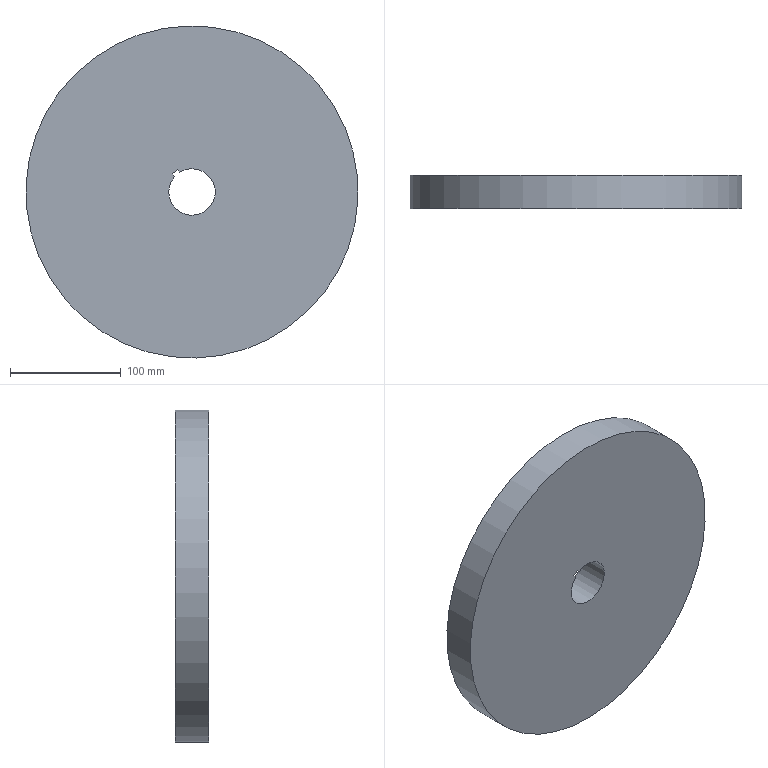Component | NX | MODEL1 | 1 solid | 7 faces | box 300 x 30 x 300 mm | volume 2078459 mm3 | plane 5 | cylinder 2 | commonest cylinder face diameters 300 x1 42 x1
STEP:
#1=CARTESIAN_POINT('',(0.,0.,0.));
#2=DIRECTION('',(0.,0.,1.));
#3=DIRECTION('',(1.,0.,0.));
#4=AXIS2_PLACEMENT_3D('',#1,#2,#3);
#5=CARTESIAN_POINT('',(844.342,50.431,-88.771));
#6=VERTEX_POINT('',#5);
#7=CARTESIAN_POINT('',(842.275,50.431,-86.308));
#8=VERTEX_POINT('',#7);
#9=CARTESIAN_POINT('',(844.342,50.431,-88.771));
#10=DIRECTION('',(-0.6428,0.,0.766));
#11=VECTOR('',#10,1.);
#12=LINE('',#9,#11);
#13=CARTESIAN_POINT('',(844.342,20.431,-88.771));
#14=DIRECTION('',(-0.766,0.,-0.6428));
#15=DIRECTION('',(0.6428,0.,-0.766));
#16=AXIS2_PLACEMENT_3D('',#13,#14,#15);
#17=PLANE('',#16);
#18=CARTESIAN_POINT('',(0.,-30.));
#19=DIRECTION('',(-1.,0.));
#20=VECTOR('',#19,1.);
#21=LINE('',#18,#20);
#22=(GEOMETRIC_REPRESENTATION_CONTEXT(2)PARAMETRIC_REPRESENTATION_CONTEXT()REPRESENTATION_CONTEXT('',''));
#23=DEFINITIONAL_REPRESENTATION('',(#21),#22);
#24=PCURVE('',#17,#23);
#25=CARTESIAN_POINT('',(860.,50.431,-102.764));
#26=DIRECTION('',(0.,-1.,0.));
#27=DIRECTION('',(0.766,0.,0.6428));
#28=AXIS2_PLACEMENT_3D('',#25,#26,#27);
#29=PLANE('',#28);
#30=CARTESIAN_POINT('',(-3.,20.785));
#31=DIRECTION('',(0.,1.));
#32=VECTOR('',#31,1.);
#33=LINE('',#30,#32);
#34=(GEOMETRIC_REPRESENTATION_CONTEXT(2)PARAMETRIC_REPRESENTATION_CONTEXT()REPRESENTATION_CONTEXT('',''));
#35=DEFINITIONAL_REPRESENTATION('',(#33),#34);
#36=PCURVE('',#29,#35);
#37=SURFACE_CURVE('',#12,(#24,#36),.PCURVE_S1.);
#38=EDGE_CURVE('',#6,#8,#37,.T.);
#39=ORIENTED_EDGE('',*,*,#38,.T.);
#40=CARTESIAN_POINT('',(842.275,20.431,-86.308));
#41=VERTEX_POINT('',#40);
#42=CARTESIAN_POINT('',(842.275,20.431,-86.308));
#43=DIRECTION('',(0.,1.,0.));
#44=VECTOR('',#43,1.);
#45=LINE('',#42,#44);
#46=CARTESIAN_POINT('',(-3.215,0.));
#47=DIRECTION('',(0.,-1.));
#48=VECTOR('',#47,1.);
#49=LINE('',#46,#48);
#50=(GEOMETRIC_REPRESENTATION_CONTEXT(2)PARAMETRIC_REPRESENTATION_CONTEXT()REPRESENTATION_CONTEXT('',''));
#51=DEFINITIONAL_REPRESENTATION('',(#49),#50);
#52=PCURVE('',#17,#51);
#53=CARTESIAN_POINT('',(842.275,20.431,-86.308));
#54=DIRECTION('',(-0.6428,0.,0.766));
#55=DIRECTION('',(-0.766,0.,-0.6428));
#56=AXIS2_PLACEMENT_3D('',#53,#54,#55);
#57=PLANE('',#56);
#58=CARTESIAN_POINT('',(0.,0.));
#59=DIRECTION('',(0.,-1.));
#60=VECTOR('',#59,1.);
#61=LINE('',#58,#60);
#62=(GEOMETRIC_REPRESENTATION_CONTEXT(2)PARAMETRIC_REPRESENTATION_CONTEXT()REPRESENTATION_CONTEXT('',''));
#63=DEFINITIONAL_REPRESENTATION('',(#61),#62);
#64=PCURVE('',#57,#63);
#65=SURFACE_CURVE('',#45,(#52,#64),.PCURVE_S1.);
#66=EDGE_CURVE('',#41,#8,#65,.T.);
#67=ORIENTED_EDGE('',*,*,#66,.F.);
#68=CARTESIAN_POINT('',(844.342,20.431,-88.771));
#69=VERTEX_POINT('',#68);
#70=CARTESIAN_POINT('',(844.342,20.431,-88.771));
#71=DIRECTION('',(-0.6428,0.,0.766));
#72=VECTOR('',#71,1.);
#73=LINE('',#70,#72);
#74=CARTESIAN_POINT('',(0.,0.));
#75=DIRECTION('',(-1.,0.));
#76=VECTOR('',#75,1.);
#77=LINE('',#74,#76);
#78=(GEOMETRIC_REPRESENTATION_CONTEXT(2)PARAMETRIC_REPRESENTATION_CONTEXT()REPRESENTATION_CONTEXT('',''));
#79=DEFINITIONAL_REPRESENTATION('',(#77),#78);
#80=PCURVE('',#17,#79);
#81=CARTESIAN_POINT('',(860.,20.431,-102.764));
#82=DIRECTION('',(0.,-1.,0.));
#83=DIRECTION('',(0.766,0.,0.6428));
#84=AXIS2_PLACEMENT_3D('',#81,#82,#83);
#85=PLANE('',#84);
#86=CARTESIAN_POINT('',(-3.,20.785));
#87=DIRECTION('',(0.,1.));
#88=VECTOR('',#87,1.);
#89=LINE('',#86,#88);
#90=(GEOMETRIC_REPRESENTATION_CONTEXT(2)PARAMETRIC_REPRESENTATION_CONTEXT()REPRESENTATION_CONTEXT('',''));
#91=DEFINITIONAL_REPRESENTATION('',(#89),#90);
#92=PCURVE('',#85,#91);
#93=SURFACE_CURVE('',#73,(#80,#92),.PCURVE_S1.);
#94=EDGE_CURVE('',#69,#41,#93,.T.);
#95=ORIENTED_EDGE('',*,*,#94,.F.);
#96=CARTESIAN_POINT('',(844.342,20.431,-88.771));
#97=DIRECTION('',(0.,1.,0.));
#98=VECTOR('',#97,1.);
#99=LINE('',#96,#98);
#100=CARTESIAN_POINT('',(0.,0.));
#101=DIRECTION('',(0.,-1.));
#102=VECTOR('',#101,1.);
#103=LINE('',#100,#102);
#104=(GEOMETRIC_REPRESENTATION_CONTEXT(2)PARAMETRIC_REPRESENTATION_CONTEXT()REPRESENTATION_CONTEXT('',''));
#105=DEFINITIONAL_REPRESENTATION('',(#103),#104);
#106=PCURVE('',#17,#105);
#107=CARTESIAN_POINT('',(860.,20.431,-102.764));
#108=DIRECTION('',(0.,1.,0.));
#109=DIRECTION('',(-0.766,0.,-0.6428));
#110=AXIS2_PLACEMENT_3D('',#107,#108,#109);
#111=CYLINDRICAL_SURFACE('',#110,21.);
#112=CARTESIAN_POINT('',(7.711,0.));
#113=DIRECTION('',(0.,1.));
#114=VECTOR('',#113,1.);
#115=LINE('',#112,#114);
#116=(GEOMETRIC_REPRESENTATION_CONTEXT(2)PARAMETRIC_REPRESENTATION_CONTEXT()REPRESENTATION_CONTEXT('',''));
#117=DEFINITIONAL_REPRESENTATION('',(#115),#116);
#118=PCURVE('',#111,#117);
#119=SURFACE_CURVE('',#99,(#106,#118),.PCURVE_S1.);
#120=EDGE_CURVE('',#69,#6,#119,.T.);
#121=ORIENTED_EDGE('',*,*,#120,.T.);
#122=EDGE_LOOP('',(#39,#67,#95,#121));
#123=FACE_BOUND('',#122,.T.);
#124=ADVANCED_FACE('',(#123),#17,.F.);
#125=CARTESIAN_POINT('',(846.871,50.431,-82.451));
#126=VERTEX_POINT('',#125);
#127=CARTESIAN_POINT('',(842.275,50.431,-86.308));
#128=DIRECTION('',(0.766,0.,0.6428));
#129=VECTOR('',#128,1.);
#130=LINE('',#127,#129);
#131=CARTESIAN_POINT('',(0.,-30.));
#132=DIRECTION('',(-1.,0.));
#133=VECTOR('',#132,1.);
#134=LINE('',#131,#133);
#135=(GEOMETRIC_REPRESENTATION_CONTEXT(2)PARAMETRIC_REPRESENTATION_CONTEXT()REPRESENTATION_CONTEXT('',''));
#136=DEFINITIONAL_REPRESENTATION('',(#134),#135);
#137=PCURVE('',#57,#136);
#138=CARTESIAN_POINT('',(-3.,24.));
#139=DIRECTION('',(1.,-0.));
#140=VECTOR('',#139,1.);
#141=LINE('',#138,#140);
#142=(GEOMETRIC_REPRESENTATION_CONTEXT(2)PARAMETRIC_REPRESENTATION_CONTEXT()REPRESENTATION_CONTEXT('',''));
#143=DEFINITIONAL_REPRESENTATION('',(#141),#142);
#144=PCURVE('',#29,#143);
#145=SURFACE_CURVE('',#130,(#137,#144),.PCURVE_S1.);
#146=EDGE_CURVE('',#8,#126,#145,.T.);
#147=ORIENTED_EDGE('',*,*,#146,.T.);
#148=CARTESIAN_POINT('',(846.871,20.431,-82.451));
#149=VERTEX_POINT('',#148);
#150=CARTESIAN_POINT('',(846.871,20.431,-82.451));
#151=DIRECTION('',(0.,1.,0.));
#152=VECTOR('',#151,1.);
#153=LINE('',#150,#152);
#154=CARTESIAN_POINT('',(-6.,0.));
#155=DIRECTION('',(0.,-1.));
#156=VECTOR('',#155,1.);
#157=LINE('',#154,#156);
#158=(GEOMETRIC_REPRESENTATION_CONTEXT(2)PARAMETRIC_REPRESENTATION_CONTEXT()REPRESENTATION_CONTEXT('',''));
#159=DEFINITIONAL_REPRESENTATION('',(#157),#158);
#160=PCURVE('',#57,#159);
#161=CARTESIAN_POINT('',(846.871,20.431,-82.451));
#162=DIRECTION('',(0.766,0.,0.6428));
#163=DIRECTION('',(-0.6428,0.,0.766));
#164=AXIS2_PLACEMENT_3D('',#161,#162,#163);
#165=PLANE('',#164);
#166=CARTESIAN_POINT('',(-0.,0.));
#167=DIRECTION('',(0.,-1.));
#168=VECTOR('',#167,1.);
#169=LINE('',#166,#168);
#170=(GEOMETRIC_REPRESENTATION_CONTEXT(2)PARAMETRIC_REPRESENTATION_CONTEXT()REPRESENTATION_CONTEXT('',''));
#171=DEFINITIONAL_REPRESENTATION('',(#169),#170);
#172=PCURVE('',#165,#171);
#173=SURFACE_CURVE('',#153,(#160,#172),.PCURVE_S1.);
#174=EDGE_CURVE('',#149,#126,#173,.T.);
#175=ORIENTED_EDGE('',*,*,#174,.F.);
#176=CARTESIAN_POINT('',(842.275,20.431,-86.308));
#177=DIRECTION('',(0.766,0.,0.6428));
#178=VECTOR('',#177,1.);
#179=LINE('',#176,#178);
#180=CARTESIAN_POINT('',(0.,0.));
#181=DIRECTION('',(-1.,0.));
#182=VECTOR('',#181,1.);
#183=LINE('',#180,#182);
#184=(GEOMETRIC_REPRESENTATION_CONTEXT(2)PARAMETRIC_REPRESENTATION_CONTEXT()REPRESENTATION_CONTEXT('',''));
#185=DEFINITIONAL_REPRESENTATION('',(#183),#184);
#186=PCURVE('',#57,#185);
#187=CARTESIAN_POINT('',(-3.,24.));
#188=DIRECTION('',(1.,-0.));
#189=VECTOR('',#188,1.);
#190=LINE('',#187,#189);
#191=(GEOMETRIC_REPRESENTATION_CONTEXT(2)PARAMETRIC_REPRESENTATION_CONTEXT()REPRESENTATION_CONTEXT('',''));
#192=DEFINITIONAL_REPRESENTATION('',(#190),#191);
#193=PCURVE('',#85,#192);
#194=SURFACE_CURVE('',#179,(#186,#193),.PCURVE_S1.);
#195=EDGE_CURVE('',#41,#149,#194,.T.);
#196=ORIENTED_EDGE('',*,*,#195,.F.);
#197=ORIENTED_EDGE('',*,*,#66,.T.);
#198=EDGE_LOOP('',(#147,#175,#196,#197));
#199=FACE_BOUND('',#198,.T.);
#200=ADVANCED_FACE('',(#199),#57,.F.);
#201=CARTESIAN_POINT('',(848.938,50.431,-84.914));
#202=VERTEX_POINT('',#201);
#203=CARTESIAN_POINT('',(846.871,50.431,-82.451));
#204=DIRECTION('',(0.6428,0.,-0.766));
#205=VECTOR('',#204,1.);
#206=LINE('',#203,#205);
#207=CARTESIAN_POINT('',(0.,-30.));
#208=DIRECTION('',(-1.,0.));
#209=VECTOR('',#208,1.);
#210=LINE('',#207,#209);
#211=(GEOMETRIC_REPRESENTATION_CONTEXT(2)PARAMETRIC_REPRESENTATION_CONTEXT()REPRESENTATION_CONTEXT('',''));
#212=DEFINITIONAL_REPRESENTATION('',(#210),#211);
#213=PCURVE('',#165,#212);
#214=CARTESIAN_POINT('',(3.,24.));
#215=DIRECTION('',(0.,-1.));
#216=VECTOR('',#215,1.);
#217=LINE('',#214,#216);
#218=(GEOMETRIC_REPRESENTATION_CONTEXT(2)PARAMETRIC_REPRESENTATION_CONTEXT()REPRESENTATION_CONTEXT('',''));
#219=DEFINITIONAL_REPRESENTATION('',(#217),#218);
#220=PCURVE('',#29,#219);
#221=SURFACE_CURVE('',#206,(#213,#220),.PCURVE_S1.);
#222=EDGE_CURVE('',#126,#202,#221,.T.);
#223=ORIENTED_EDGE('',*,*,#222,.T.);
#224=CARTESIAN_POINT('',(848.938,20.431,-84.914));
#225=VERTEX_POINT('',#224);
#226=CARTESIAN_POINT('',(848.938,20.431,-84.914));
#227=DIRECTION('',(0.,1.,0.));
#228=VECTOR('',#227,1.);
#229=LINE('',#226,#228);
#230=CARTESIAN_POINT('',(-3.215,0.));
#231=DIRECTION('',(0.,-1.));
#232=VECTOR('',#231,1.);
#233=LINE('',#230,#232);
#234=(GEOMETRIC_REPRESENTATION_CONTEXT(2)PARAMETRIC_REPRESENTATION_CONTEXT()REPRESENTATION_CONTEXT('',''));
#235=DEFINITIONAL_REPRESENTATION('',(#233),#234);
#236=PCURVE('',#165,#235);
#237=CARTESIAN_POINT('',(1.714,0.));
#238=DIRECTION('',(0.,1.));
#239=VECTOR('',#238,1.);
#240=LINE('',#237,#239);
#241=(GEOMETRIC_REPRESENTATION_CONTEXT(2)PARAMETRIC_REPRESENTATION_CONTEXT()REPRESENTATION_CONTEXT('',''));
#242=DEFINITIONAL_REPRESENTATION('',(#240),#241);
#243=PCURVE('',#111,#242);
#244=SURFACE_CURVE('',#229,(#236,#243),.PCURVE_S1.);
#245=EDGE_CURVE('',#225,#202,#244,.T.);
#246=ORIENTED_EDGE('',*,*,#245,.F.);
#247=CARTESIAN_POINT('',(846.871,20.431,-82.451));
#248=DIRECTION('',(0.6428,0.,-0.766));
#249=VECTOR('',#248,1.);
#250=LINE('',#247,#249);
#251=CARTESIAN_POINT('',(0.,0.));
#252=DIRECTION('',(-1.,0.));
#253=VECTOR('',#252,1.);
#254=LINE('',#251,#253);
#255=(GEOMETRIC_REPRESENTATION_CONTEXT(2)PARAMETRIC_REPRESENTATION_CONTEXT()REPRESENTATION_CONTEXT('',''));
#256=DEFINITIONAL_REPRESENTATION('',(#254),#255);
#257=PCURVE('',#165,#256);
#258=CARTESIAN_POINT('',(3.,24.));
#259=DIRECTION('',(0.,-1.));
#260=VECTOR('',#259,1.);
#261=LINE('',#258,#260);
#262=(GEOMETRIC_REPRESENTATION_CONTEXT(2)PARAMETRIC_REPRESENTATION_CONTEXT()REPRESENTATION_CONTEXT('',''));
#263=DEFINITIONAL_REPRESENTATION('',(#261),#262);
#264=PCURVE('',#85,#263);
#265=SURFACE_CURVE('',#250,(#257,#264),.PCURVE_S1.);
#266=EDGE_CURVE('',#149,#225,#265,.T.);
#267=ORIENTED_EDGE('',*,*,#266,.F.);
#268=ORIENTED_EDGE('',*,*,#174,.T.);
#269=EDGE_LOOP('',(#223,#246,#267,#268));
#270=FACE_BOUND('',#269,.T.);
#271=ADVANCED_FACE('',(#270),#165,.F.);
#272=CARTESIAN_POINT('',(974.907,20.431,-6.346));
#273=VERTEX_POINT('',#272);
#274=CARTESIAN_POINT('',(860.,20.431,-102.764));
#275=DIRECTION('',(0.,-1.,0.));
#276=DIRECTION('',(0.766,0.,0.6428));
#277=AXIS2_PLACEMENT_3D('',#274,#275,#276);
#278=CIRCLE('',#277,150.);
#279=CARTESIAN_POINT('',(860.,20.431,-102.764));
#280=DIRECTION('',(0.,1.,0.));
#281=DIRECTION('',(-0.766,0.,-0.6428));
#282=AXIS2_PLACEMENT_3D('',#279,#280,#281);
#283=CYLINDRICAL_SURFACE('',#282,150.);
#284=CARTESIAN_POINT('',(9.425,0.));
#285=DIRECTION('',(-1.,0.));
#286=VECTOR('',#285,1.);
#287=LINE('',#284,#286);
#288=(GEOMETRIC_REPRESENTATION_CONTEXT(2)PARAMETRIC_REPRESENTATION_CONTEXT()REPRESENTATION_CONTEXT('',''));
#289=DEFINITIONAL_REPRESENTATION('',(#287),#288);
#290=PCURVE('',#283,#289);
#291=CARTESIAN_POINT('',(0.,0.));
#292=DIRECTION('',(1.,0.));
#293=AXIS2_PLACEMENT_2D('',#291,#292);
#294=CIRCLE('',#293,150.);
#295=(GEOMETRIC_REPRESENTATION_CONTEXT(2)PARAMETRIC_REPRESENTATION_CONTEXT()REPRESENTATION_CONTEXT('',''));
#296=DEFINITIONAL_REPRESENTATION('',(#294),#295);
#297=PCURVE('',#85,#296);
#298=SURFACE_CURVE('',#278,(#290,#297),.PCURVE_S1.);
#299=EDGE_CURVE('',#273,#273,#298,.T.);
#300=ORIENTED_EDGE('',*,*,#299,.F.);
#301=CARTESIAN_POINT('',(974.907,50.431,-6.346));
#302=VERTEX_POINT('',#301);
#303=CARTESIAN_POINT('',(974.907,20.431,-6.346));
#304=CARTESIAN_POINT('',(974.907,50.431,-6.346));
#305=B_SPLINE_CURVE_WITH_KNOTS('',1,(#303,#304),.UNSPECIFIED.,.F.,.F.,(2,2),(0.,30.),.PIECEWISE_BEZIER_KNOTS.);
#306=CARTESIAN_POINT('',(9.425,0.));
#307=DIRECTION('',(0.,1.));
#308=VECTOR('',#307,1.);
#309=LINE('',#306,#308);
#310=(GEOMETRIC_REPRESENTATION_CONTEXT(2)PARAMETRIC_REPRESENTATION_CONTEXT()REPRESENTATION_CONTEXT('',''));
#311=DEFINITIONAL_REPRESENTATION('',(#309),#310);
#312=PCURVE('',#283,#311);
#313=CARTESIAN_POINT('',(3.142,0.));
#314=DIRECTION('',(0.,1.));
#315=VECTOR('',#314,1.);
#316=LINE('',#313,#315);
#317=(GEOMETRIC_REPRESENTATION_CONTEXT(2)PARAMETRIC_REPRESENTATION_CONTEXT()REPRESENTATION_CONTEXT('',''));
#318=DEFINITIONAL_REPRESENTATION('',(#316),#317);
#319=PCURVE('',#283,#318);
#320=SEAM_CURVE('',#305,(#312,#319),.PCURVE_S1.);
#321=EDGE_CURVE('',#273,#302,#320,.T.);
#322=ORIENTED_EDGE('',*,*,#321,.T.);
#323=CARTESIAN_POINT('',(860.,50.431,-102.764));
#324=DIRECTION('',(0.,-1.,0.));
#325=DIRECTION('',(0.766,0.,0.6428));
#326=AXIS2_PLACEMENT_3D('',#323,#324,#325);
#327=CIRCLE('',#326,150.);
#328=CARTESIAN_POINT('',(9.425,30.));
#329=DIRECTION('',(-1.,0.));
#330=VECTOR('',#329,1.);
#331=LINE('',#328,#330);
#332=(GEOMETRIC_REPRESENTATION_CONTEXT(2)PARAMETRIC_REPRESENTATION_CONTEXT()REPRESENTATION_CONTEXT('',''));
#333=DEFINITIONAL_REPRESENTATION('',(#331),#332);
#334=PCURVE('',#283,#333);
#335=CARTESIAN_POINT('',(0.,0.));
#336=DIRECTION('',(1.,0.));
#337=AXIS2_PLACEMENT_2D('',#335,#336);
#338=CIRCLE('',#337,150.);
#339=(GEOMETRIC_REPRESENTATION_CONTEXT(2)PARAMETRIC_REPRESENTATION_CONTEXT()REPRESENTATION_CONTEXT('',''));
#340=DEFINITIONAL_REPRESENTATION('',(#338),#339);
#341=PCURVE('',#29,#340);
#342=SURFACE_CURVE('',#327,(#334,#341),.PCURVE_S1.);
#343=EDGE_CURVE('',#302,#302,#342,.T.);
#344=ORIENTED_EDGE('',*,*,#343,.T.);
#345=ORIENTED_EDGE('',*,*,#321,.F.);
#346=EDGE_LOOP('',(#300,#322,#344,#345));
#347=FACE_BOUND('',#346,.T.);
#348=ADVANCED_FACE('',(#347),#283,.T.);
#349=ORIENTED_EDGE('',*,*,#245,.F.);
#350=CARTESIAN_POINT('',(860.,20.431,-102.764));
#351=DIRECTION('',(0.,1.,0.));
#352=DIRECTION('',(0.766,0.,0.6428));
#353=AXIS2_PLACEMENT_3D('',#350,#351,#352);
#354=CIRCLE('',#353,21.);
#355=CARTESIAN_POINT('',(-3.142,0.));
#356=DIRECTION('',(1.,0.));
#357=VECTOR('',#356,1.);
#358=LINE('',#355,#357);
#359=(GEOMETRIC_REPRESENTATION_CONTEXT(2)PARAMETRIC_REPRESENTATION_CONTEXT()REPRESENTATION_CONTEXT('',''));
#360=DEFINITIONAL_REPRESENTATION('',(#358),#359);
#361=PCURVE('',#111,#360);
#362=CARTESIAN_POINT('',(21.,0.));
#363=CARTESIAN_POINT('',(21.,-36.373));
#364=CARTESIAN_POINT('',(-10.5,-18.187));
#365=CARTESIAN_POINT('',(-42.,-0.));
#366=CARTESIAN_POINT('',(-10.5,18.187));
#367=CARTESIAN_POINT('',(21.,36.373));
#368=CARTESIAN_POINT('',(21.,0.));
#369=(BOUNDED_CURVE()B_SPLINE_CURVE(2,(#362,#363,#364,#365,#366,#367,#368),.UNSPECIFIED.,.T.,.F.)B_SPLINE_CURVE_WITH_KNOTS((1,2,2,2,2,1),(-2.094,0.,2.094,4.189,6.283,8.378),.UNSPECIFIED.)CURVE()GEOMETRIC_REPRESENTATION_ITEM()RATIONAL_B_SPLINE_CURVE((1.,0.5,1.,0.5,1.,0.5,1.))REPRESENTATION_ITEM(''));
#370=(GEOMETRIC_REPRESENTATION_CONTEXT(2)PARAMETRIC_REPRESENTATION_CONTEXT()REPRESENTATION_CONTEXT('',''));
#371=DEFINITIONAL_REPRESENTATION('',(#369),#370);
#372=PCURVE('',#85,#371);
#373=SURFACE_CURVE('',#354,(#361,#372),.PCURVE_S1.);
#374=EDGE_CURVE('',#225,#69,#373,.T.);
#375=ORIENTED_EDGE('',*,*,#374,.T.);
#376=ORIENTED_EDGE('',*,*,#120,.T.);
#377=CARTESIAN_POINT('',(860.,50.431,-102.764));
#378=DIRECTION('',(0.,1.,0.));
#379=DIRECTION('',(0.766,0.,0.6428));
#380=AXIS2_PLACEMENT_3D('',#377,#378,#379);
#381=CIRCLE('',#380,21.);
#382=CARTESIAN_POINT('',(-3.142,30.));
#383=DIRECTION('',(1.,0.));
#384=VECTOR('',#383,1.);
#385=LINE('',#382,#384);
#386=(GEOMETRIC_REPRESENTATION_CONTEXT(2)PARAMETRIC_REPRESENTATION_CONTEXT()REPRESENTATION_CONTEXT('',''));
#387=DEFINITIONAL_REPRESENTATION('',(#385),#386);
#388=PCURVE('',#111,#387);
#389=CARTESIAN_POINT('',(21.,0.));
#390=CARTESIAN_POINT('',(21.,-36.373));
#391=CARTESIAN_POINT('',(-10.5,-18.187));
#392=CARTESIAN_POINT('',(-42.,-0.));
#393=CARTESIAN_POINT('',(-10.5,18.187));
#394=CARTESIAN_POINT('',(21.,36.373));
#395=CARTESIAN_POINT('',(21.,0.));
#396=(BOUNDED_CURVE()B_SPLINE_CURVE(2,(#389,#390,#391,#392,#393,#394,#395),.UNSPECIFIED.,.T.,.F.)B_SPLINE_CURVE_WITH_KNOTS((1,2,2,2,2,1),(-2.094,0.,2.094,4.189,6.283,8.378),.UNSPECIFIED.)CURVE()GEOMETRIC_REPRESENTATION_ITEM()RATIONAL_B_SPLINE_CURVE((1.,0.5,1.,0.5,1.,0.5,1.))REPRESENTATION_ITEM(''));
#397=(GEOMETRIC_REPRESENTATION_CONTEXT(2)PARAMETRIC_REPRESENTATION_CONTEXT()REPRESENTATION_CONTEXT('',''));
#398=DEFINITIONAL_REPRESENTATION('',(#396),#397);
#399=PCURVE('',#29,#398);
#400=SURFACE_CURVE('',#381,(#388,#399),.PCURVE_S1.);
#401=EDGE_CURVE('',#202,#6,#400,.T.);
#402=ORIENTED_EDGE('',*,*,#401,.F.);
#403=EDGE_LOOP('',(#349,#375,#376,#402));
#404=FACE_BOUND('',#403,.F.);
#405=ADVANCED_FACE('',(#404),#111,.F.);
#406=ORIENTED_EDGE('',*,*,#299,.T.);
#407=EDGE_LOOP('',(#406));
#408=FACE_BOUND('',#407,.T.);
#409=ORIENTED_EDGE('',*,*,#94,.T.);
#410=ORIENTED_EDGE('',*,*,#195,.T.);
#411=ORIENTED_EDGE('',*,*,#266,.T.);
#412=ORIENTED_EDGE('',*,*,#374,.T.);
#413=EDGE_LOOP('',(#409,#410,#411,#412));
#414=FACE_BOUND('',#413,.T.);
#415=ADVANCED_FACE('',(#408,#414),#85,.T.);
#416=ORIENTED_EDGE('',*,*,#343,.F.);
#417=EDGE_LOOP('',(#416));
#418=FACE_BOUND('',#417,.T.);
#419=ORIENTED_EDGE('',*,*,#38,.F.);
#420=ORIENTED_EDGE('',*,*,#401,.F.);
#421=ORIENTED_EDGE('',*,*,#222,.F.);
#422=ORIENTED_EDGE('',*,*,#146,.F.);
#423=EDGE_LOOP('',(#419,#420,#421,#422));
#424=FACE_BOUND('',#423,.T.);
#425=ADVANCED_FACE('',(#418,#424),#29,.F.);
#426=CLOSED_SHELL('',(#124,#200,#271,#348,#405,#415,#425));
#427=MANIFOLD_SOLID_BREP('',#426);
#428=(LENGTH_UNIT()NAMED_UNIT(*)SI_UNIT(.MILLI.,.METRE.));
#429=UNCERTAINTY_MEASURE_WITH_UNIT(LENGTH_MEASURE(0.000002),#428,'','');
#430=(NAMED_UNIT(*)PLANE_ANGLE_UNIT()SI_UNIT($,.RADIAN.));
#431=(NAMED_UNIT(*)SI_UNIT($,.STERADIAN.)SOLID_ANGLE_UNIT());
#432=(GEOMETRIC_REPRESENTATION_CONTEXT(3)GLOBAL_UNCERTAINTY_ASSIGNED_CONTEXT((#429))GLOBAL_UNIT_ASSIGNED_CONTEXT((#428,#430,#431))REPRESENTATION_CONTEXT('',''));
#433=ADVANCED_BREP_SHAPE_REPRESENTATION('',(#4,#427),#432);